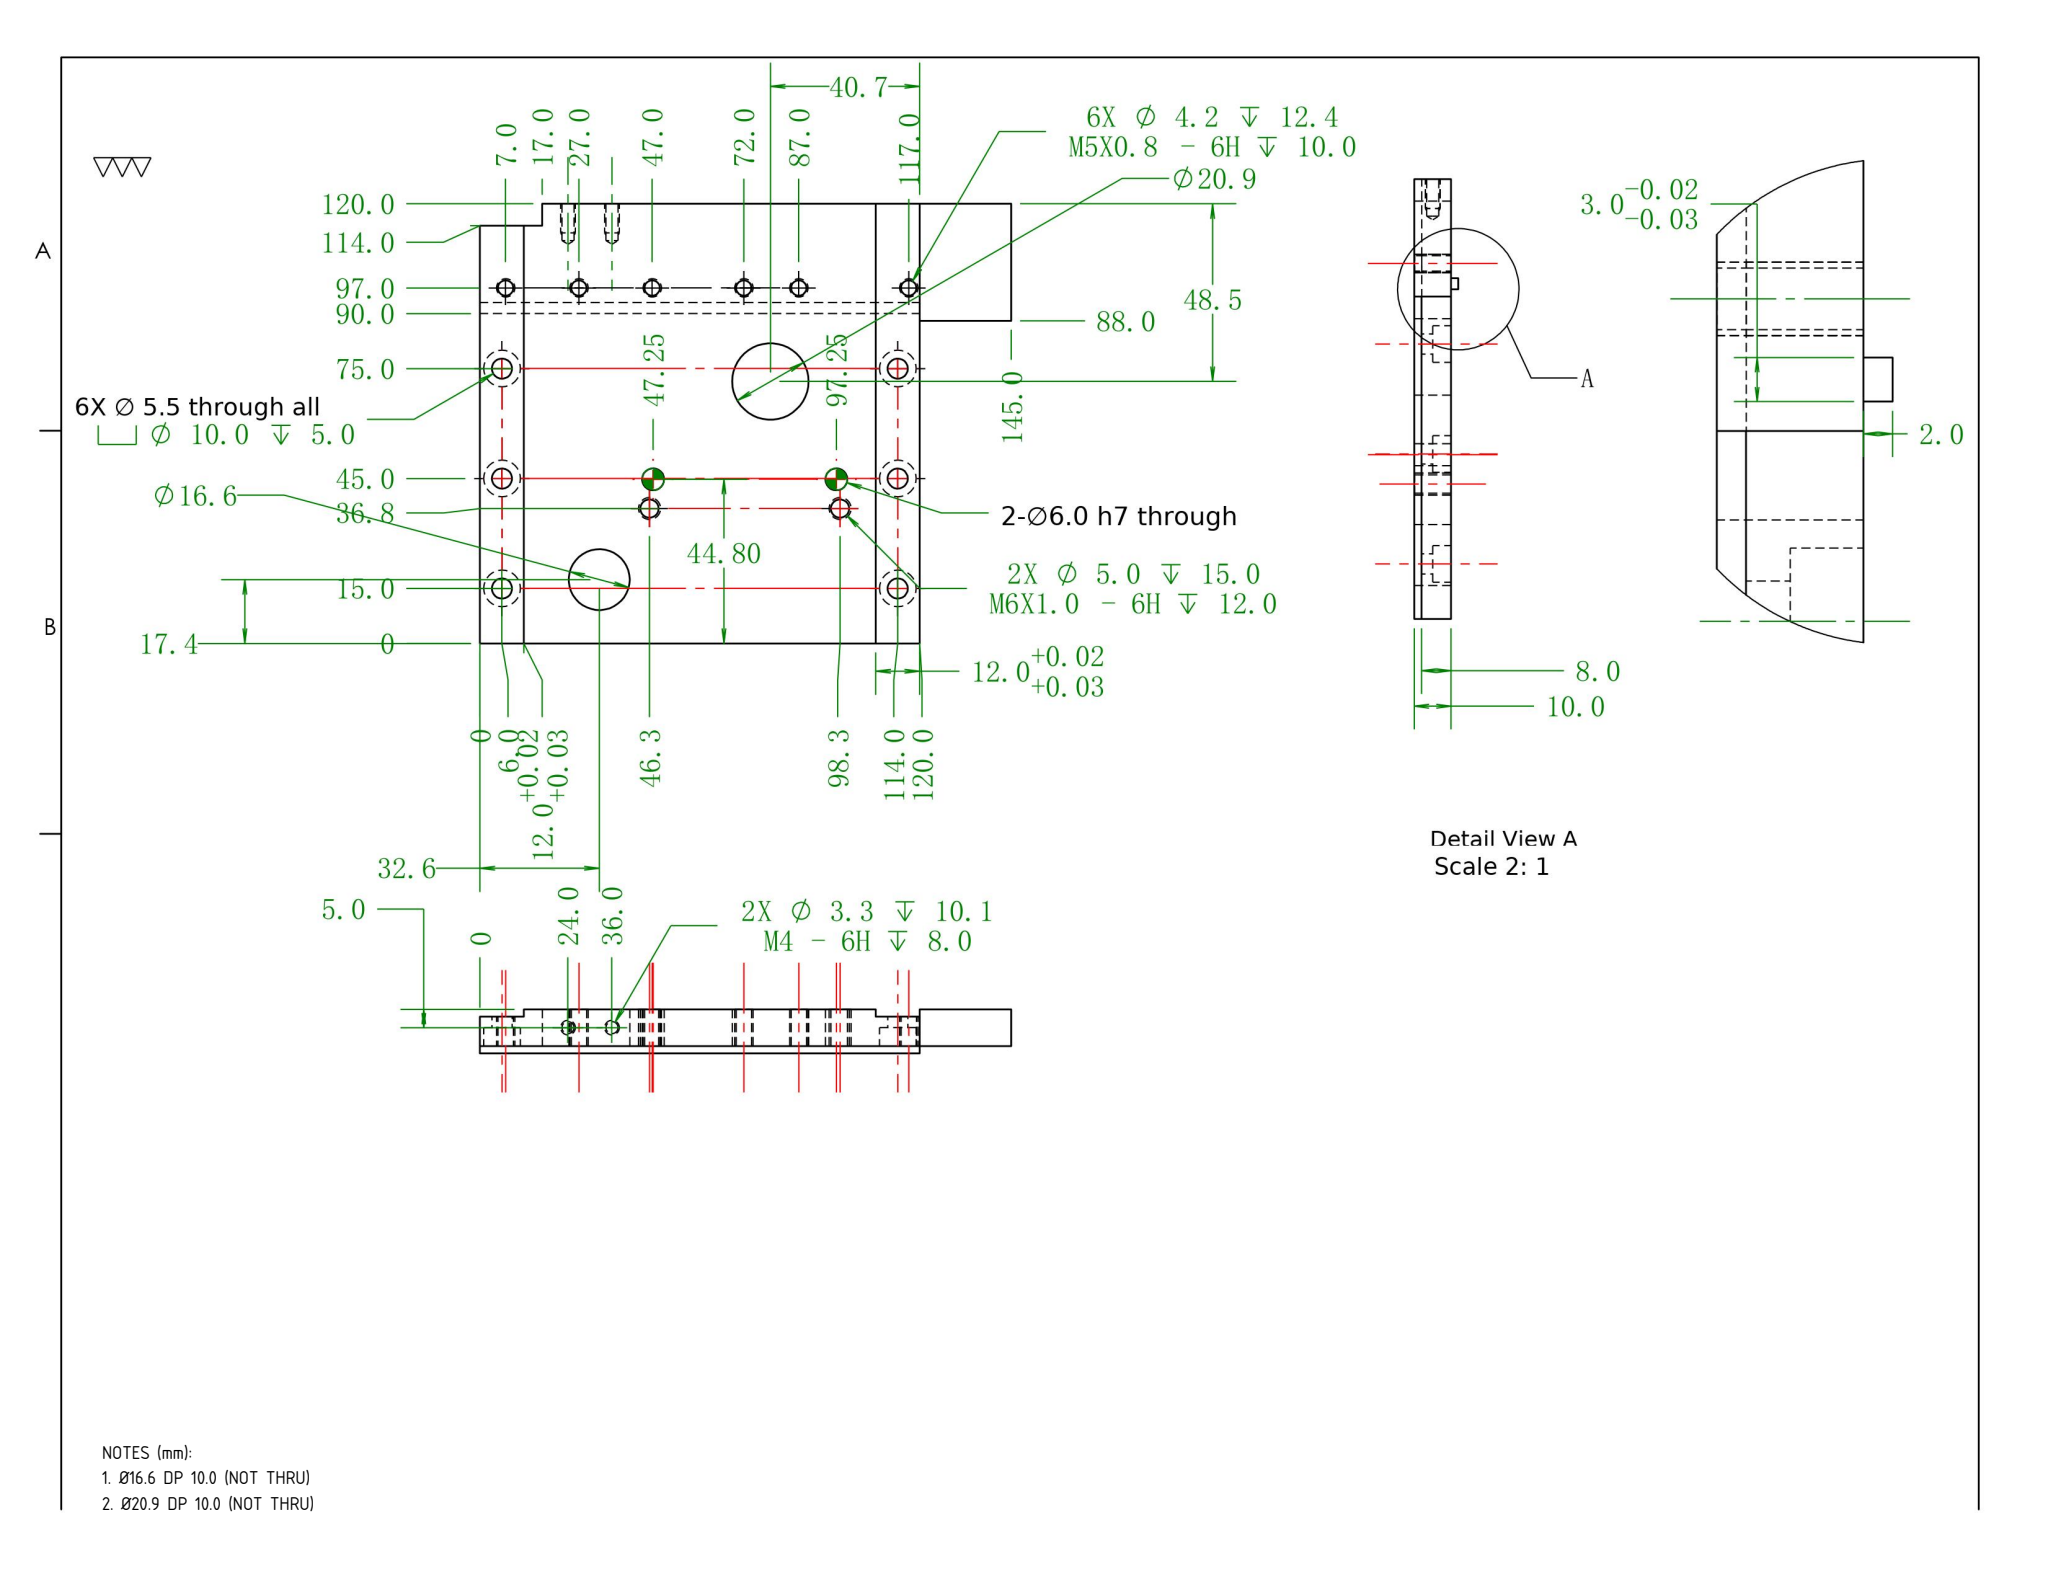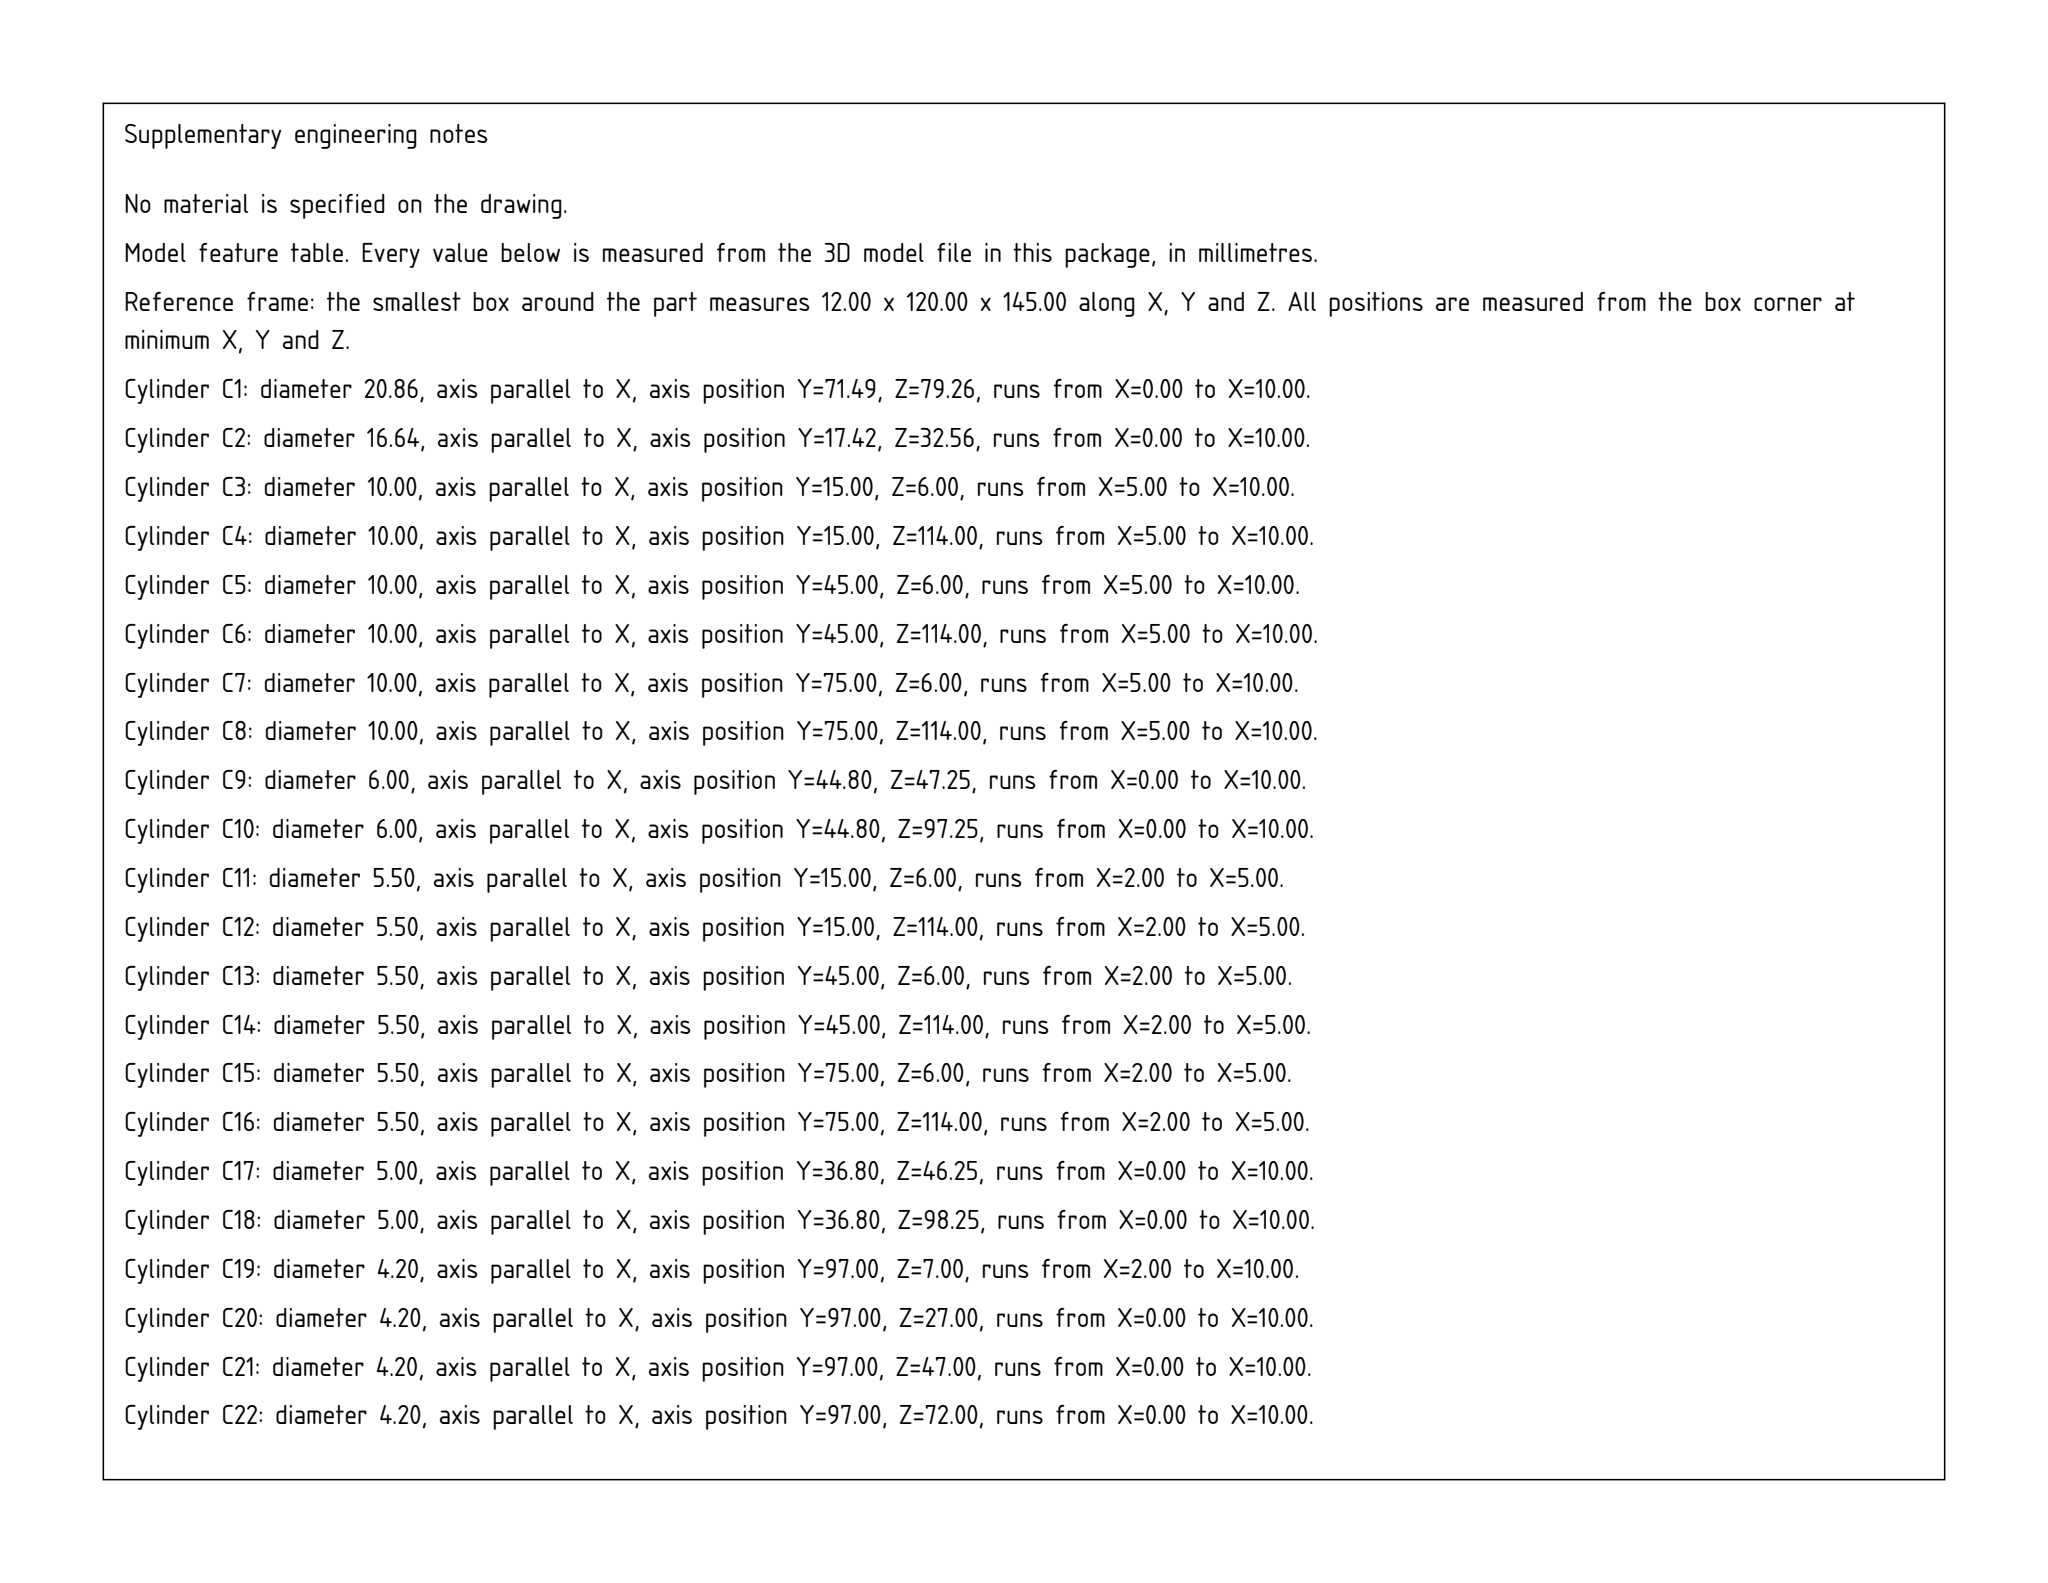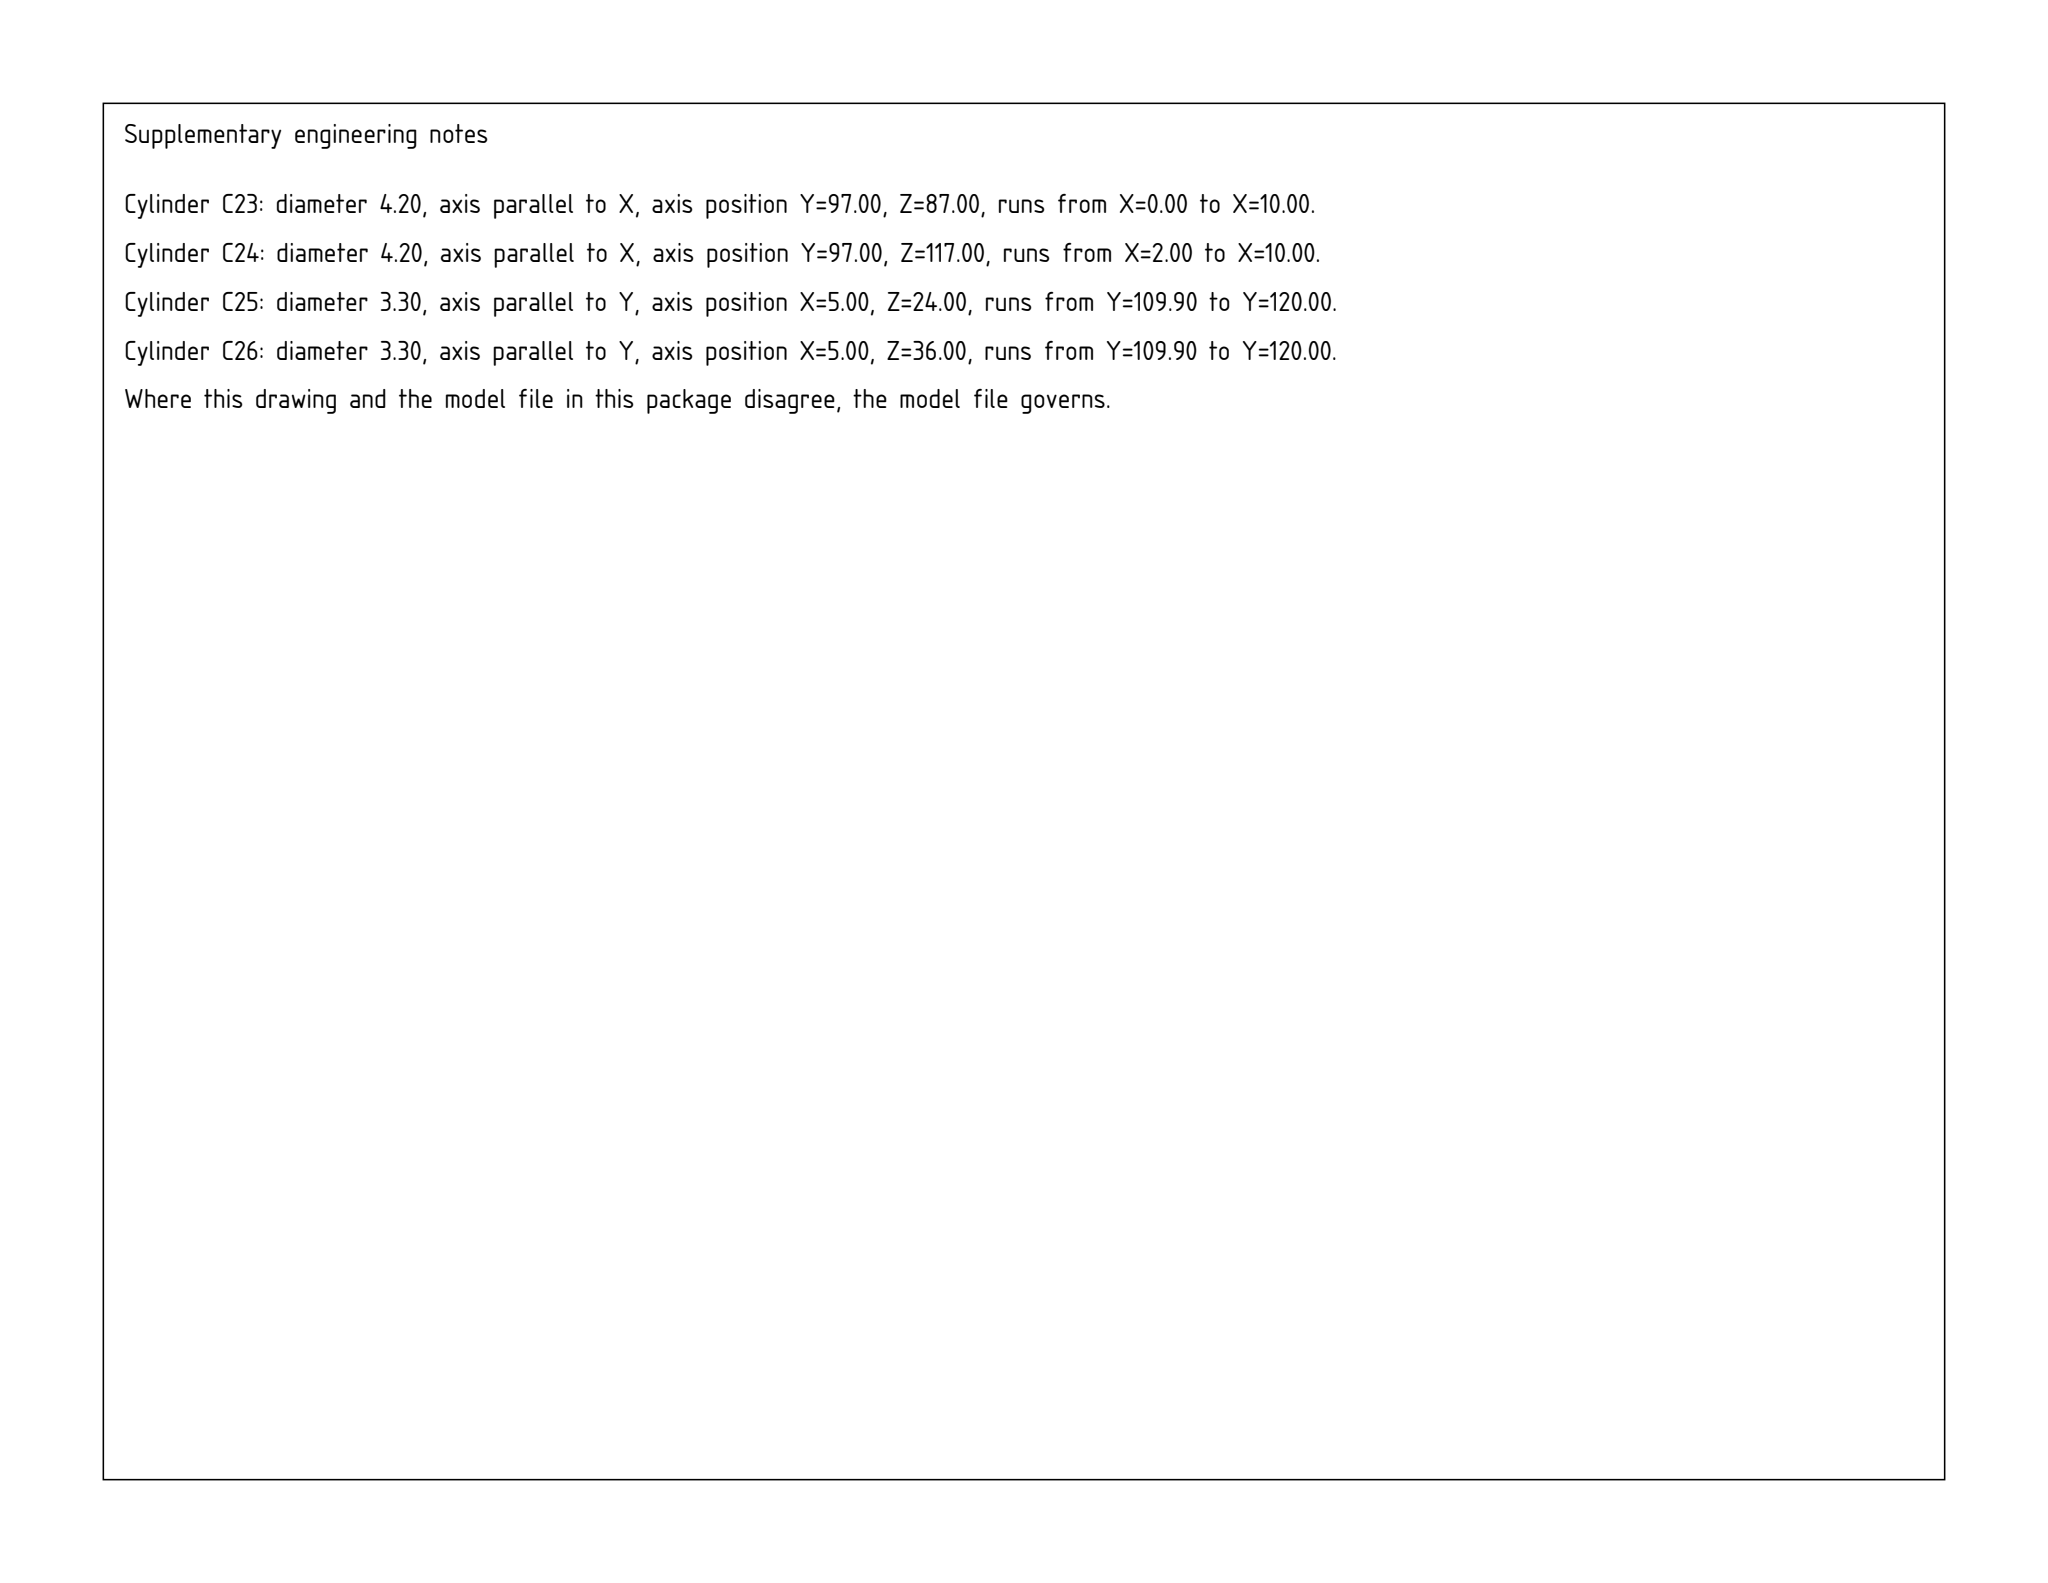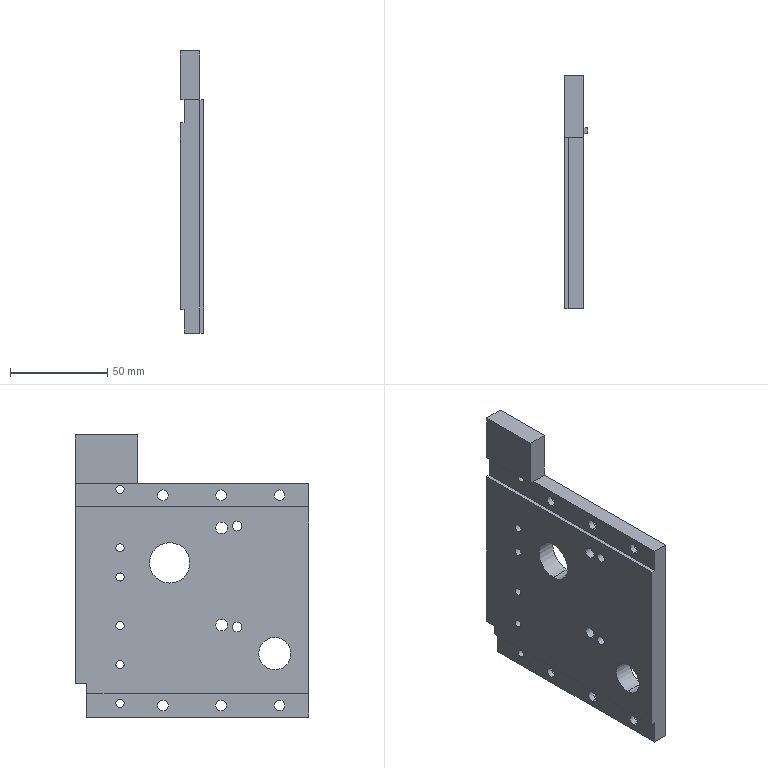Part | SolidWorks | mm | 1 solid | 82 faces | box 12 x 120 x 145 mm | volume 135800 mm3 | cylinder 52 | plane 26 | cone 4 | commonest cylinder face diameters 5.5 x12 10 x12 4.2 x12 3.3 x4 6 x4 5 x4 20.853 x2 16.632 x2
Drawing notes:
Ø16.6 DP 10.0 (NOT THRU) | from the solid: cylinder dia 16.632, axis x, length 10.0 in 12.0 thick plate
Ø20.9 DP 10.0 (NOT THRU) | from the solid: cylinder dia 20.853, axis x, length 10.0 in 12.0 thick plate
build123d program:
from build123d import *

# Parameters (mm, degrees)
SKETCH1_W                                       = 120
SKETCH1_H                                       = 80
EXTRUDE1_DEPTH                                  = 10
SKETCH2_W                                       = 120
SKETCH2_H                                       = 3
EXTRUDE2_DEPTH                                  = 2
LPATTERN1_COUNT                                 = 3
LPATTERN1_PITCH                                 = 40
SKETCH9_W                                       = 10
SKETCH9_H                                       = 22
EXTRUDE7_DEPTH                                  = 10
SKETCH10_W                                      = 10
SKETCH10_H                                      = 22
EXTRUDE8_DEPTH                                  = 15
SKETCH11_W                                      = 12
SKETCH11_H                                      = 80
EXTRUDE9_DEPTH                                  = 2
EXTRUDE10_DEPTH                                 = 40
EXTRUDE12_DEPTH                                 = 10
M6X1_0_TAPPED_HOLE1_D                           = 5
M6X1_0_TAPPED_HOLE1_DEPTH                       = 15
M6X1_0_TAPPED_HOLE1_TIP                         = 1.502
SKETCH17_R                                      = 3
CUT_EXTRUDE1_DEPTH                              = 145.568
M5X0_8_TAPPED_HOLE2_D                           = 4.2
M5X0_8_TAPPED_HOLE2_DEPTH                       = 12.4
M5X0_8_TAPPED_HOLE2_TIP                         = 1.262
M5_HEX_SOCKET_HEAD_CAP_SCREW_CBORE1_D           = 5.5
M5_HEX_SOCKET_HEAD_CAP_SCREW_CBORE1_CBORE_D     = 10
M5_HEX_SOCKET_HEAD_CAP_SCREW_CBORE1_CBORE_DEPTH = 5
LPATTERN2_COUNT                                 = 3
LPATTERN2_PITCH                                 = 30
SKETCH22_W                                      = 17
SKETCH22_H                                      = 6
CUT_EXTRUDE2_DEPTH                              = 10
M4_TAPPED_HOLE1_D                               = 3.3
M4_TAPPED_HOLE1_DEPTH                           = 10.1
M4_TAPPED_HOLE1_TIP                             = 0.9914
SKETCH25_R                                      = 10.427
SKETCH25_R_2                                    = 8.316
CUT_EXTRUDE3_DEPTH                              = 18


with BuildPart() as part:
    # Sketch1 → Extrude1 (new body)
    with BuildSketch(Plane(origin=(0, 0, 0), x_dir=(0, 0, -1), z_dir=(1, 0, 0))):
        with Locations((60, 40)):
            Rectangle(SKETCH1_W, SKETCH1_H)
    extrude(amount=EXTRUDE1_DEPTH)

    # Sketch2 → Extrude2 (add)
    with BuildSketch(Plane(origin=(10, 0, 0), x_dir=(0, 0, -1), z_dir=(1, 0, 0))):
        with Locations((60, 51.5)):
            Rectangle(SKETCH2_W, SKETCH2_H)
    extrude(amount=EXTRUDE2_DEPTH)

    # Sketch3 → M5x0.8 Tapped Hole1 (revolve, cut)
    with BuildSketch(Plane(origin=(10, 57, -33), x_dir=(0, 0, -1), z_dir=(0, 1, 0))):
        Polygon((0, 0), (0, 13.662), (2.1, 12.4), (2.1, 0), align=None)
    m5x0_8_tapped_hole1 = revolve(axis=Axis((16.35, 57, -33), (-1, 0, 0)), mode=Mode.SUBTRACT)

    # LPattern1: M5x0.8 Tapped Hole1 ×3
    with Locations(*[(0, 0, -i * LPATTERN1_PITCH) for i in range(1, LPATTERN1_COUNT)]):
        add(m5x0_8_tapped_hole1, mode=Mode.SUBTRACT)

    # Sketch9 → Extrude7 (add)
    with BuildSketch(Plane.XY):
        with Locations((5, 69)):
            Rectangle(SKETCH9_W, SKETCH9_H)
    extrude(amount=EXTRUDE7_DEPTH)

    # Sketch10 → Extrude8 (add)
    with BuildSketch(Plane.XY.offset(10)):
        with Locations((5, 69)):
            Rectangle(SKETCH10_W, SKETCH10_H)
    extrude(amount=EXTRUDE8_DEPTH)

    # Sketch11 → Extrude9 (cut)
    with BuildSketch(Plane.ZY):
        with Locations((-114, 40)):
            Rectangle(SKETCH11_W, SKETCH11_H)
        with Locations((-6, 40)):
            Rectangle(SKETCH11_W, SKETCH11_H)
    extrude(amount=-EXTRUDE9_DEPTH, mode=Mode.SUBTRACT)

    # Sketch12 → Extrude10 (add)
    with BuildSketch(Plane.XZ):
        Polygon((2, 0), (2, -12), (0, -12), (0, -108), (2, -108), (2, -120), (10, -120), (10, 0), align=None)
    extrude(amount=EXTRUDE10_DEPTH)

    # Sketch14 → Extrude12 (add)
    with BuildSketch(Plane.XZ.offset(-58)):
        Polygon((0, 0), (2, 0), (10, 0), (10, 25), (0, 25), align=None)
    extrude(amount=EXTRUDE12_DEPTH)

    # M6x1.0 Tapped Hole1
    with Locations(Plane(origin=(10, 0, 0), x_dir=(0, 0, -1), z_dir=(1, 0, 0))):
        with Locations((21.75, -3.2), (73.75, -3.2)):
            Hole(M6X1_0_TAPPED_HOLE1_D / 2, depth=M6X1_0_TAPPED_HOLE1_DEPTH)
            with Locations((0, 0, -(M6X1_0_TAPPED_HOLE1_DEPTH + M6X1_0_TAPPED_HOLE1_TIP / 2))):  # 118° drill point
                Cone(0, M6X1_0_TAPPED_HOLE1_D / 2, M6X1_0_TAPPED_HOLE1_TIP, mode=Mode.SUBTRACT)

    # Sketch17 → Cut-Extrude1 (cut, through all)
    with BuildSketch(Plane(origin=(10, 0, 0), x_dir=(0, 0, -1), z_dir=(1, 0, 0))):
        with Locations((22.75, 4.8)):
            Circle(SKETCH17_R)
        with Locations((72.75, 4.8)):
            Circle(SKETCH17_R)
    extrude(amount=-CUT_EXTRUDE1_DEPTH, mode=Mode.SUBTRACT)

    # M5x0.8 Tapped Hole2
    with Locations(Plane(origin=(10, 0, 0), x_dir=(0, 0, -1), z_dir=(1, 0, 0))):
        with Locations((3, 57), (48, 57), (93, 57)):
            Hole(M5X0_8_TAPPED_HOLE2_D / 2, depth=M5X0_8_TAPPED_HOLE2_DEPTH)
            with Locations((0, 0, -(M5X0_8_TAPPED_HOLE2_DEPTH + M5X0_8_TAPPED_HOLE2_TIP / 2))):  # 118° drill point
                Cone(0, M5X0_8_TAPPED_HOLE2_D / 2, M5X0_8_TAPPED_HOLE2_TIP, mode=Mode.SUBTRACT)

    # M5 Hex Socket Head Cap Screw CBORE1 (through all)
    with Locations(Plane(origin=(10, 0, 0), x_dir=(0, 0, -1), z_dir=(1, 0, 0))):
        with Locations((6, -25), (114, -25)):
            m5_hex_socket_head_cap_screw_cbore1 = CounterBoreHole(M5_HEX_SOCKET_HEAD_CAP_SCREW_CBORE1_D / 2, M5_HEX_SOCKET_HEAD_CAP_SCREW_CBORE1_CBORE_D / 2, M5_HEX_SOCKET_HEAD_CAP_SCREW_CBORE1_CBORE_DEPTH)

    # LPattern2: M5 Hex Socket Head Cap Screw CBORE1 ×3
    with Locations(*[(0, i * LPATTERN2_PITCH, 0) for i in range(1, LPATTERN2_COUNT)]):
        add(m5_hex_socket_head_cap_screw_cbore1, mode=Mode.SUBTRACT)

    # Sketch22 → Cut-Extrude2 (cut)
    with BuildSketch(Plane(origin=(10, 0, 0), x_dir=(0, 0, -1), z_dir=(1, 0, 0))):
        with Locations((111.5, 77)):
            Rectangle(SKETCH22_W, SKETCH22_H)
    extrude(amount=-CUT_EXTRUDE2_DEPTH, mode=Mode.SUBTRACT)

    # M4 Tapped Hole1
    with Locations(Plane(origin=(0, 80, 0), x_dir=(-1, 0, 0), z_dir=(0, 1, 0))):
        with Locations((-5, -96), (-5, -84)):
            Hole(M4_TAPPED_HOLE1_D / 2, depth=M4_TAPPED_HOLE1_DEPTH)
            with Locations((0, 0, -(M4_TAPPED_HOLE1_DEPTH + M4_TAPPED_HOLE1_TIP / 2))):  # 118° drill point
                Cone(0, M4_TAPPED_HOLE1_D / 2, M4_TAPPED_HOLE1_TIP, mode=Mode.SUBTRACT)

    # Sketch25 → Cut-Extrude3 (cut)
    with BuildSketch(Plane(origin=(10, 0, 0), x_dir=(0, 0, -1), z_dir=(1, 0, 0))):
        with Locations((40.742, 31.489)):
            Circle(SKETCH25_R)
        with Locations((87.436, -22.578)):
            Circle(SKETCH25_R_2)
    extrude(amount=-CUT_EXTRUDE3_DEPTH, mode=Mode.SUBTRACT)


solid = part.part